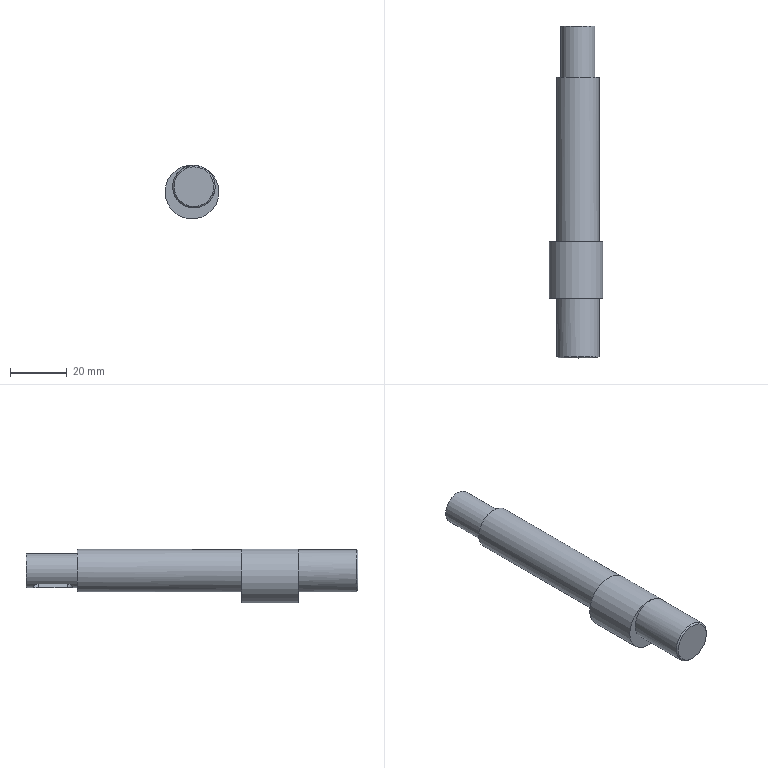Component | NX | 6 | 1 solid | 22 faces | volume 21371 mm3 | plane 10 | cylinder 8 | spline 3 | cone 1 | commonest cylinder face diameters 4 x3 15 x2 19 x1 12 x1 5 x1